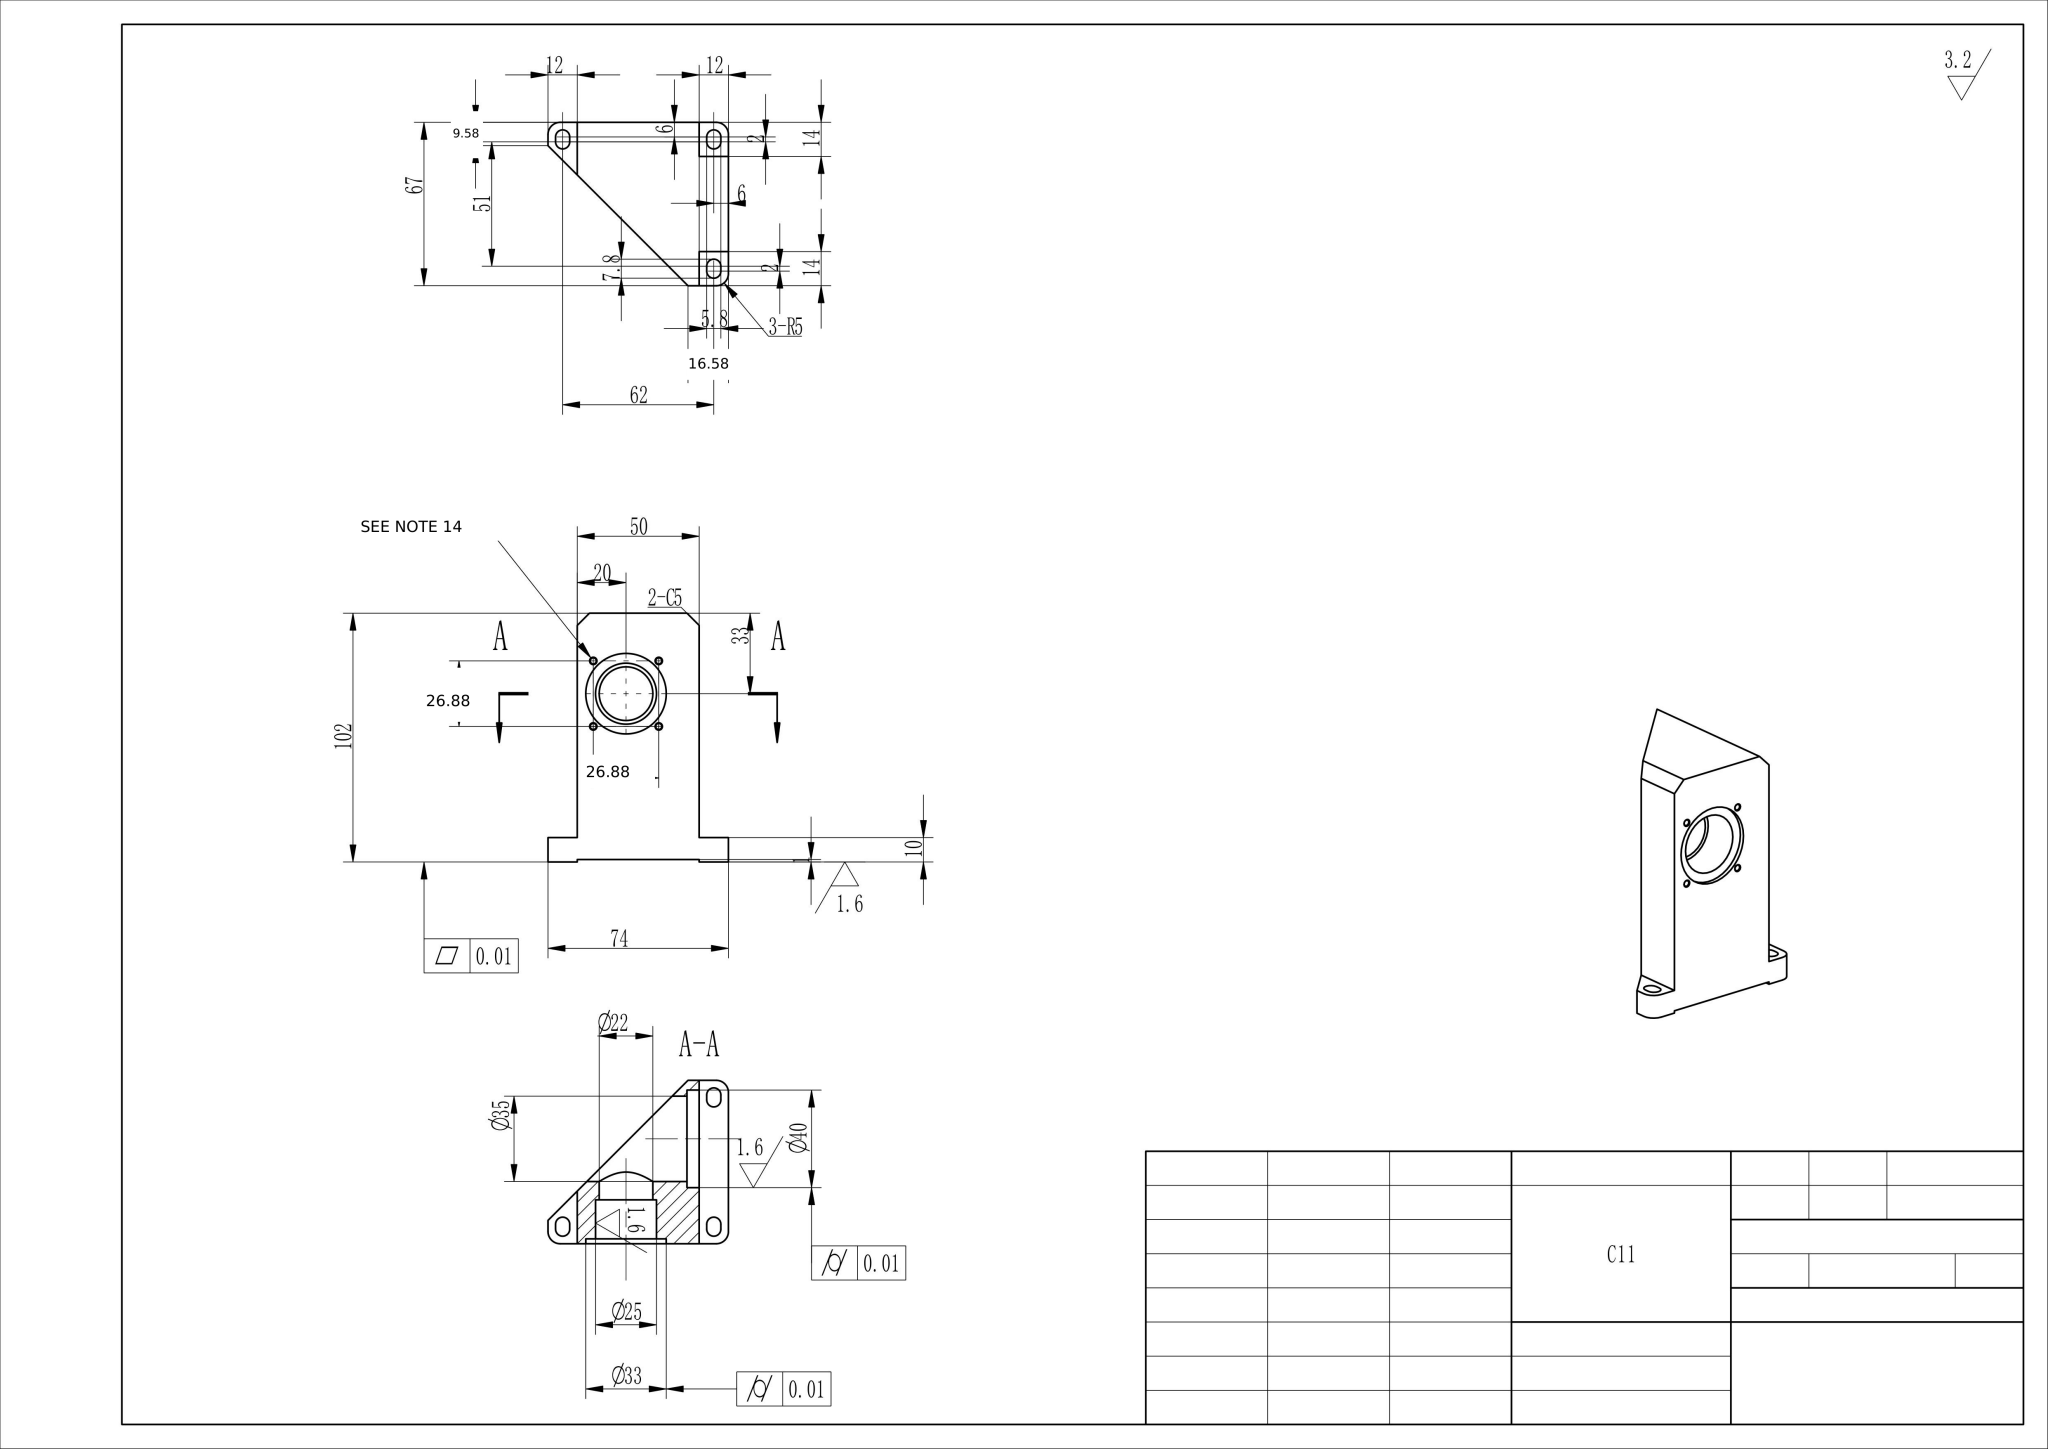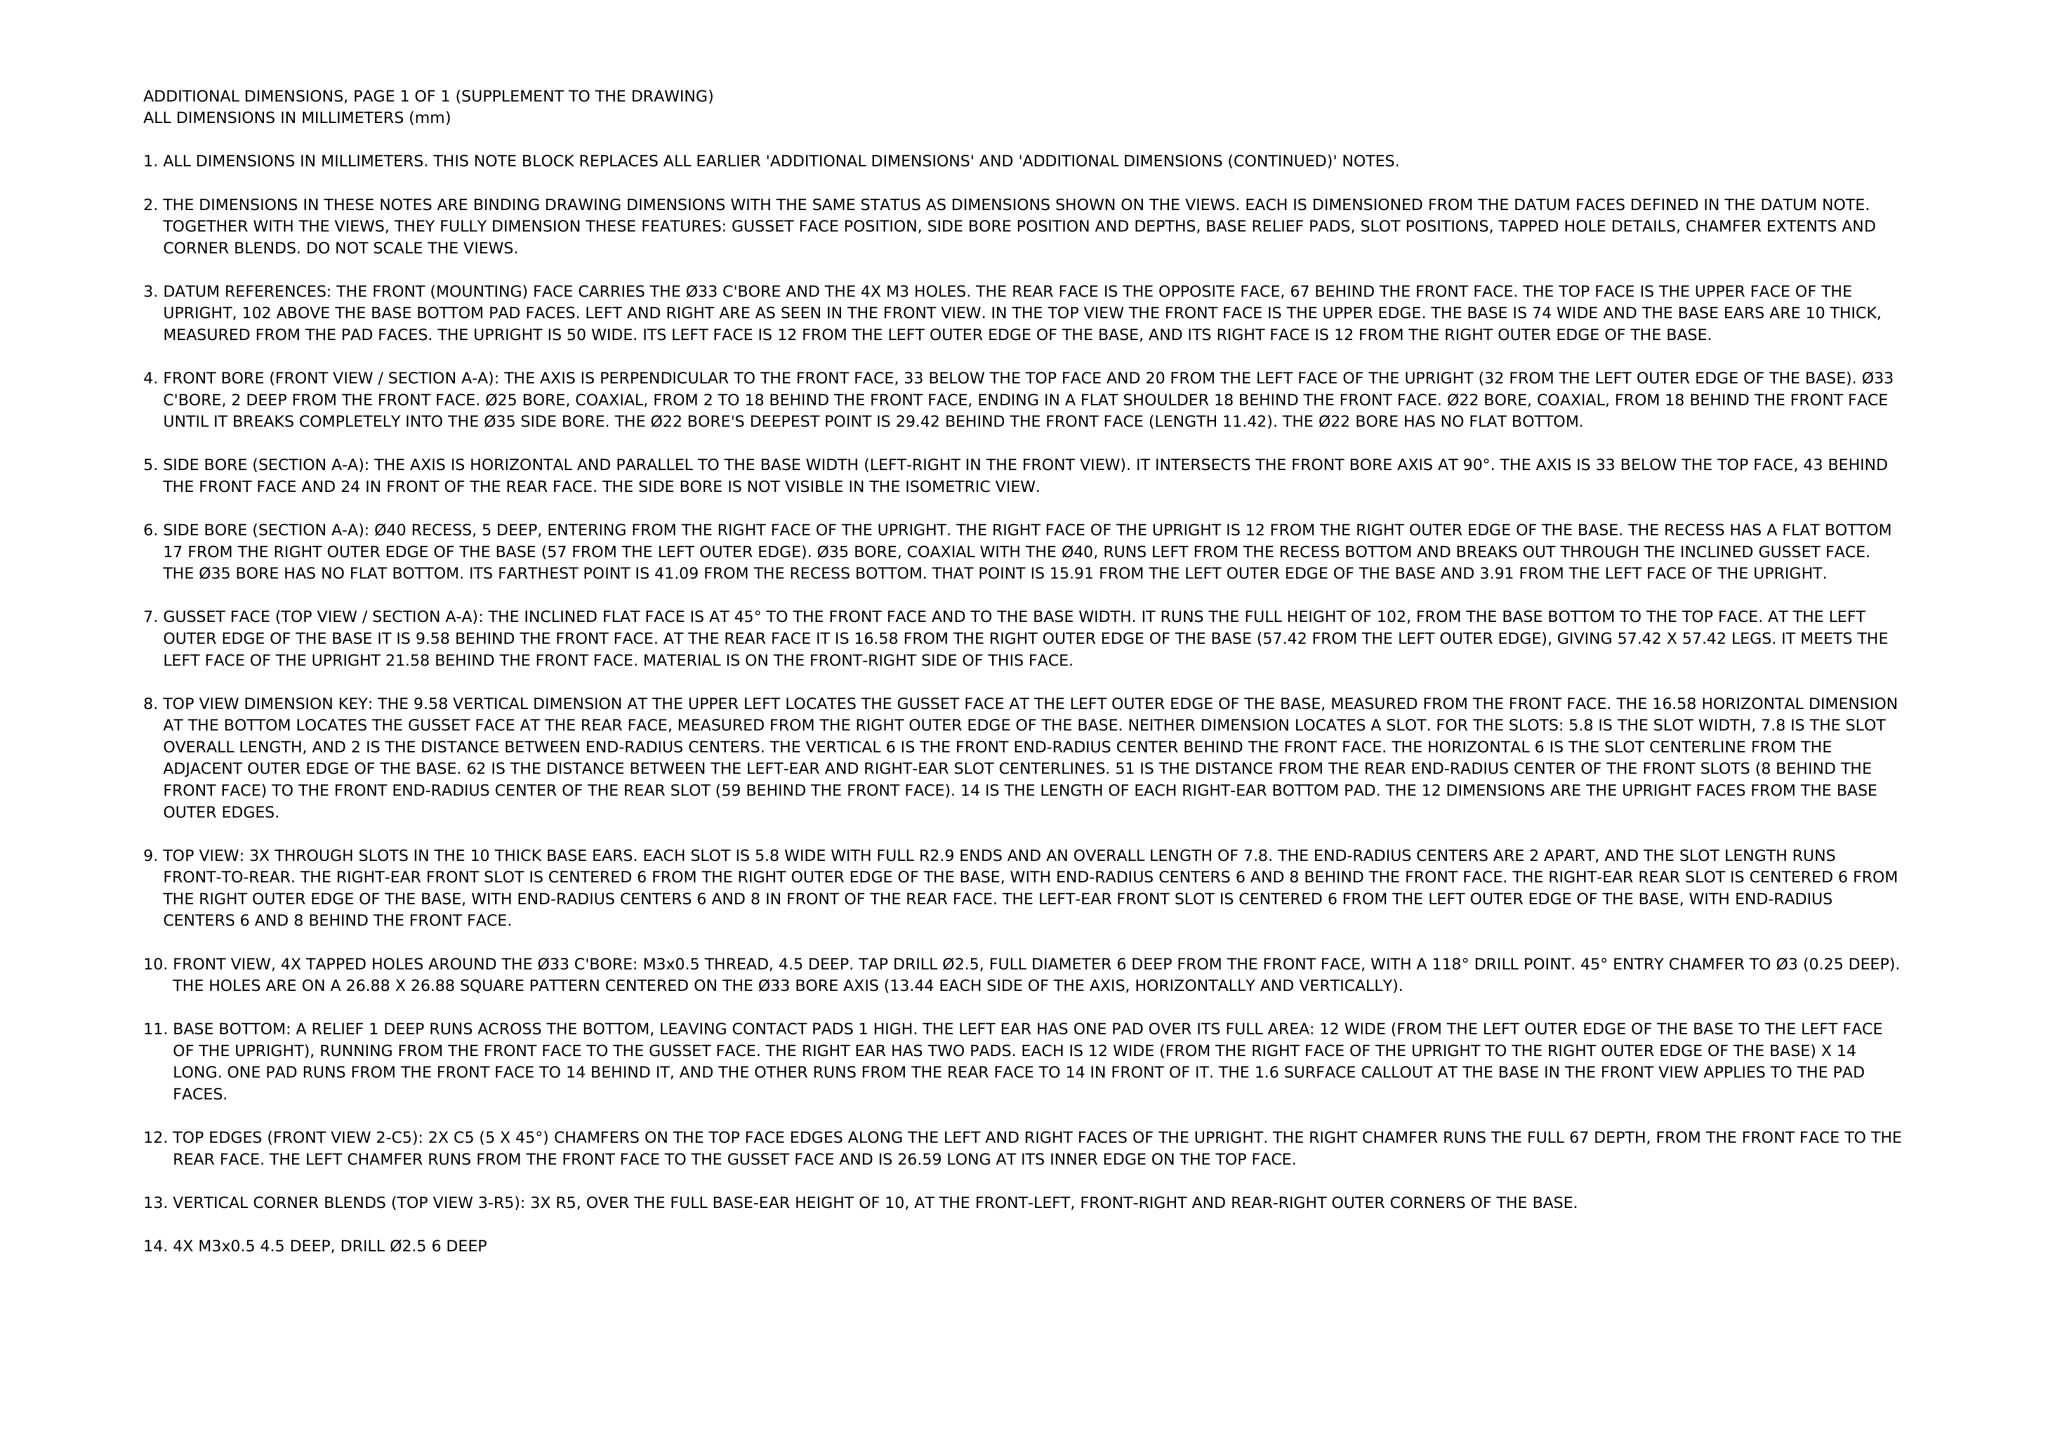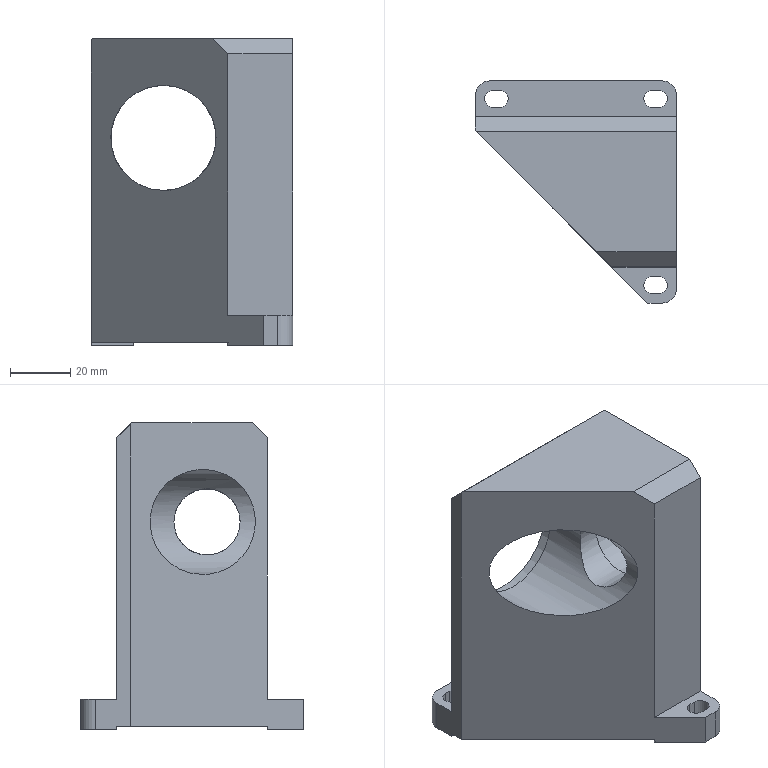Part | NX | mm | 1 solid | 56 faces | box 67 x 74 x 102 mm | volume 199346 mm3 | plane 30 | cylinder 18 | cone 8 | commonest cylinder face diameters 5.8 x6 2.5 x4 10 x3 35 x1 40 x1 22 x1 25 x1 33 x1